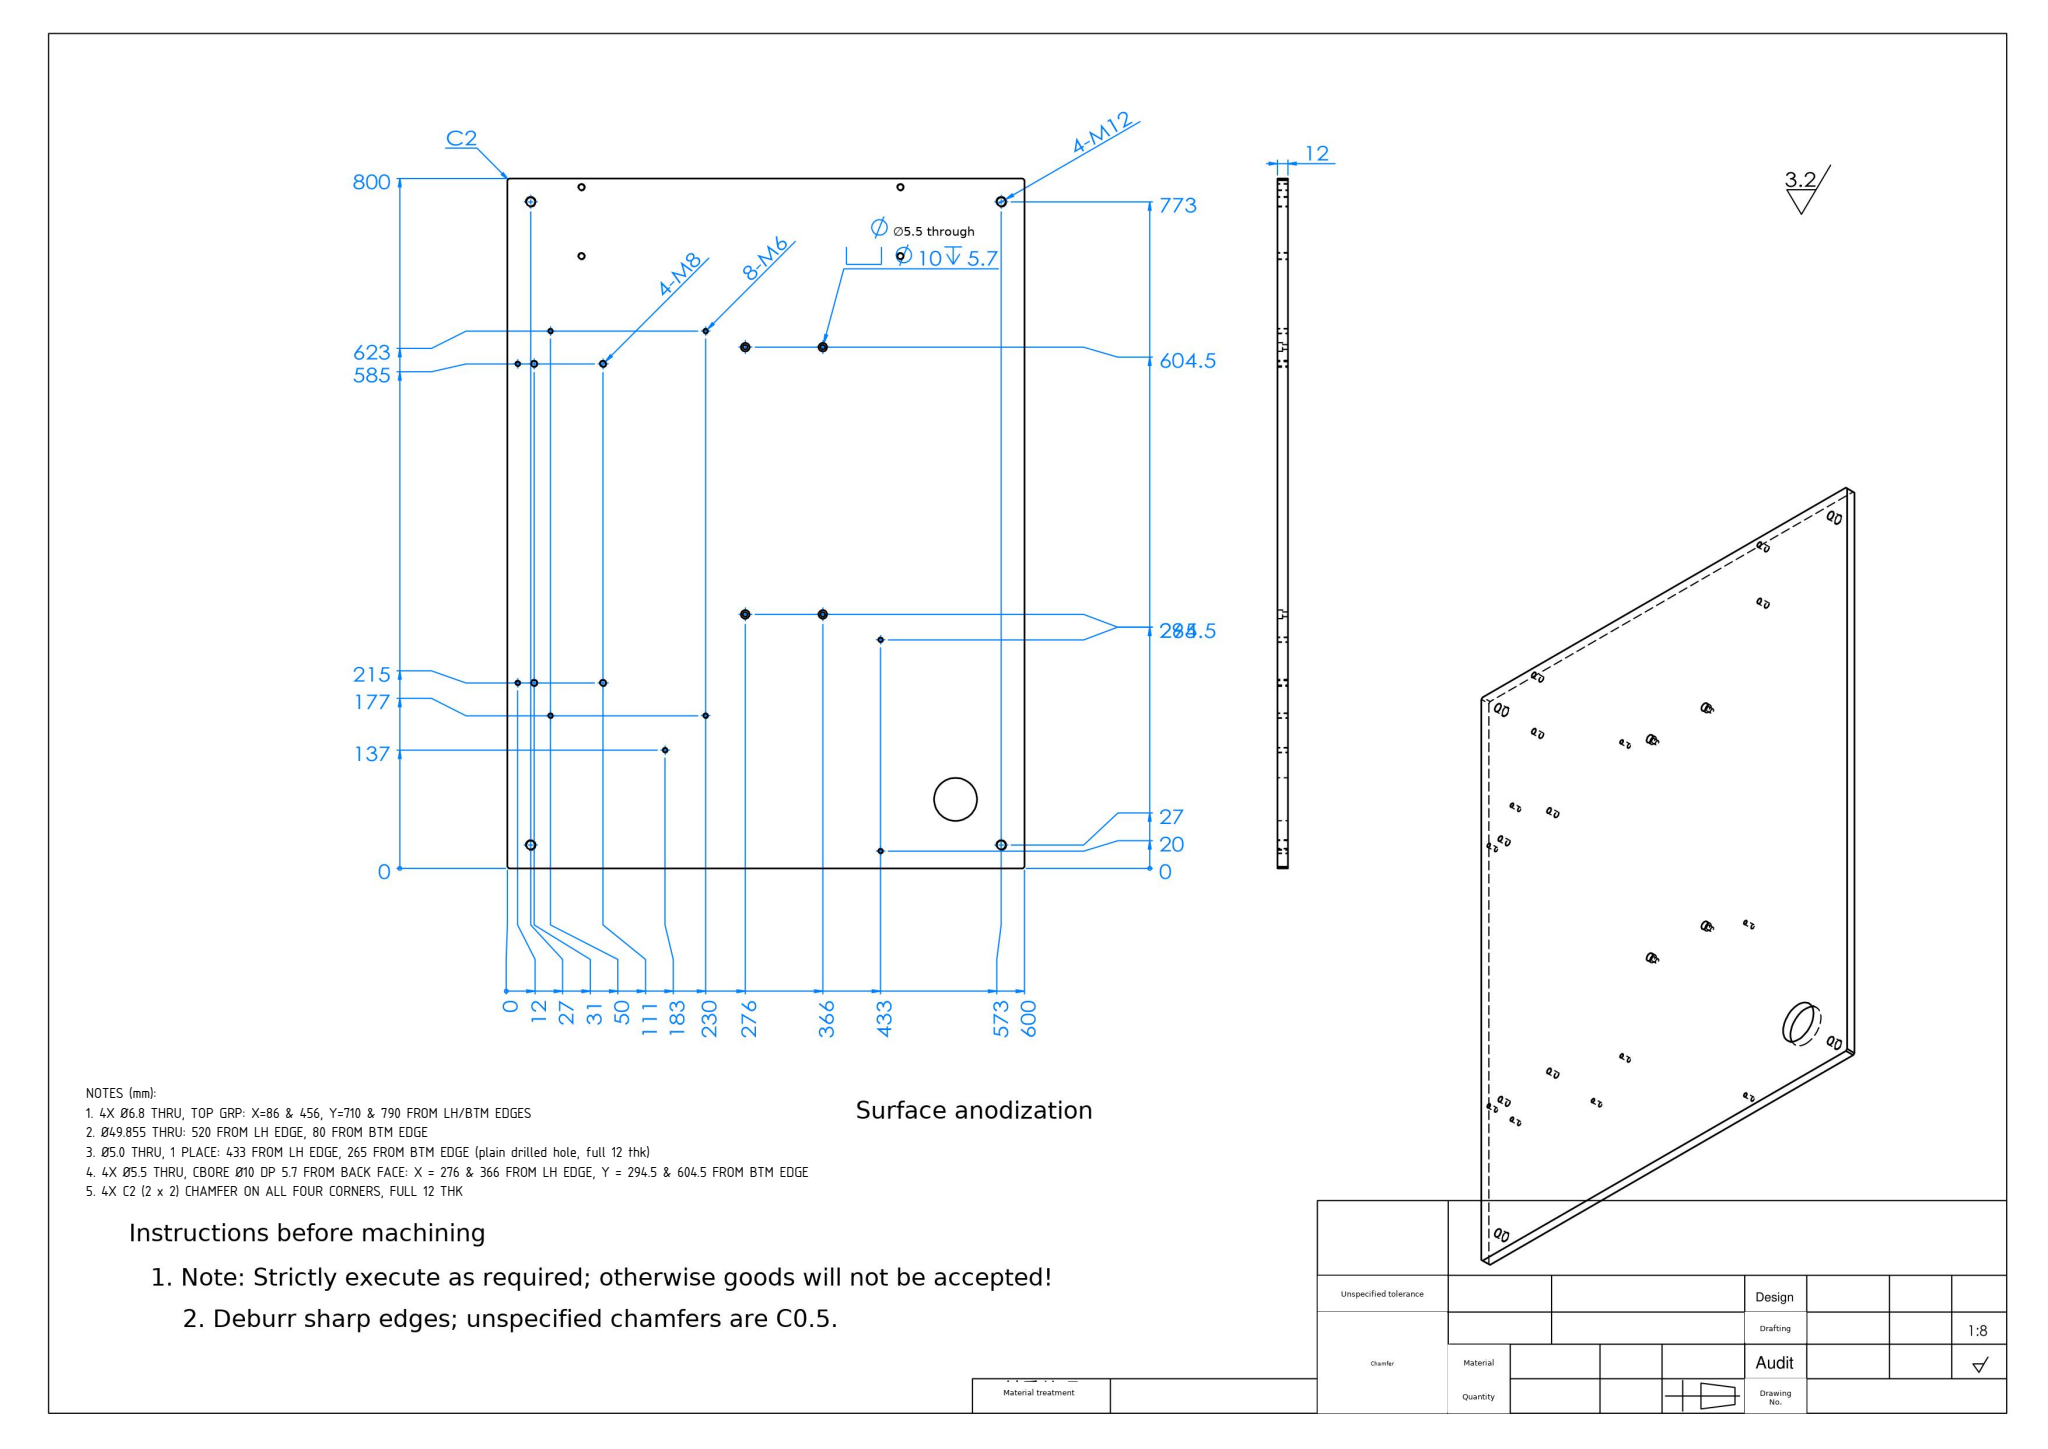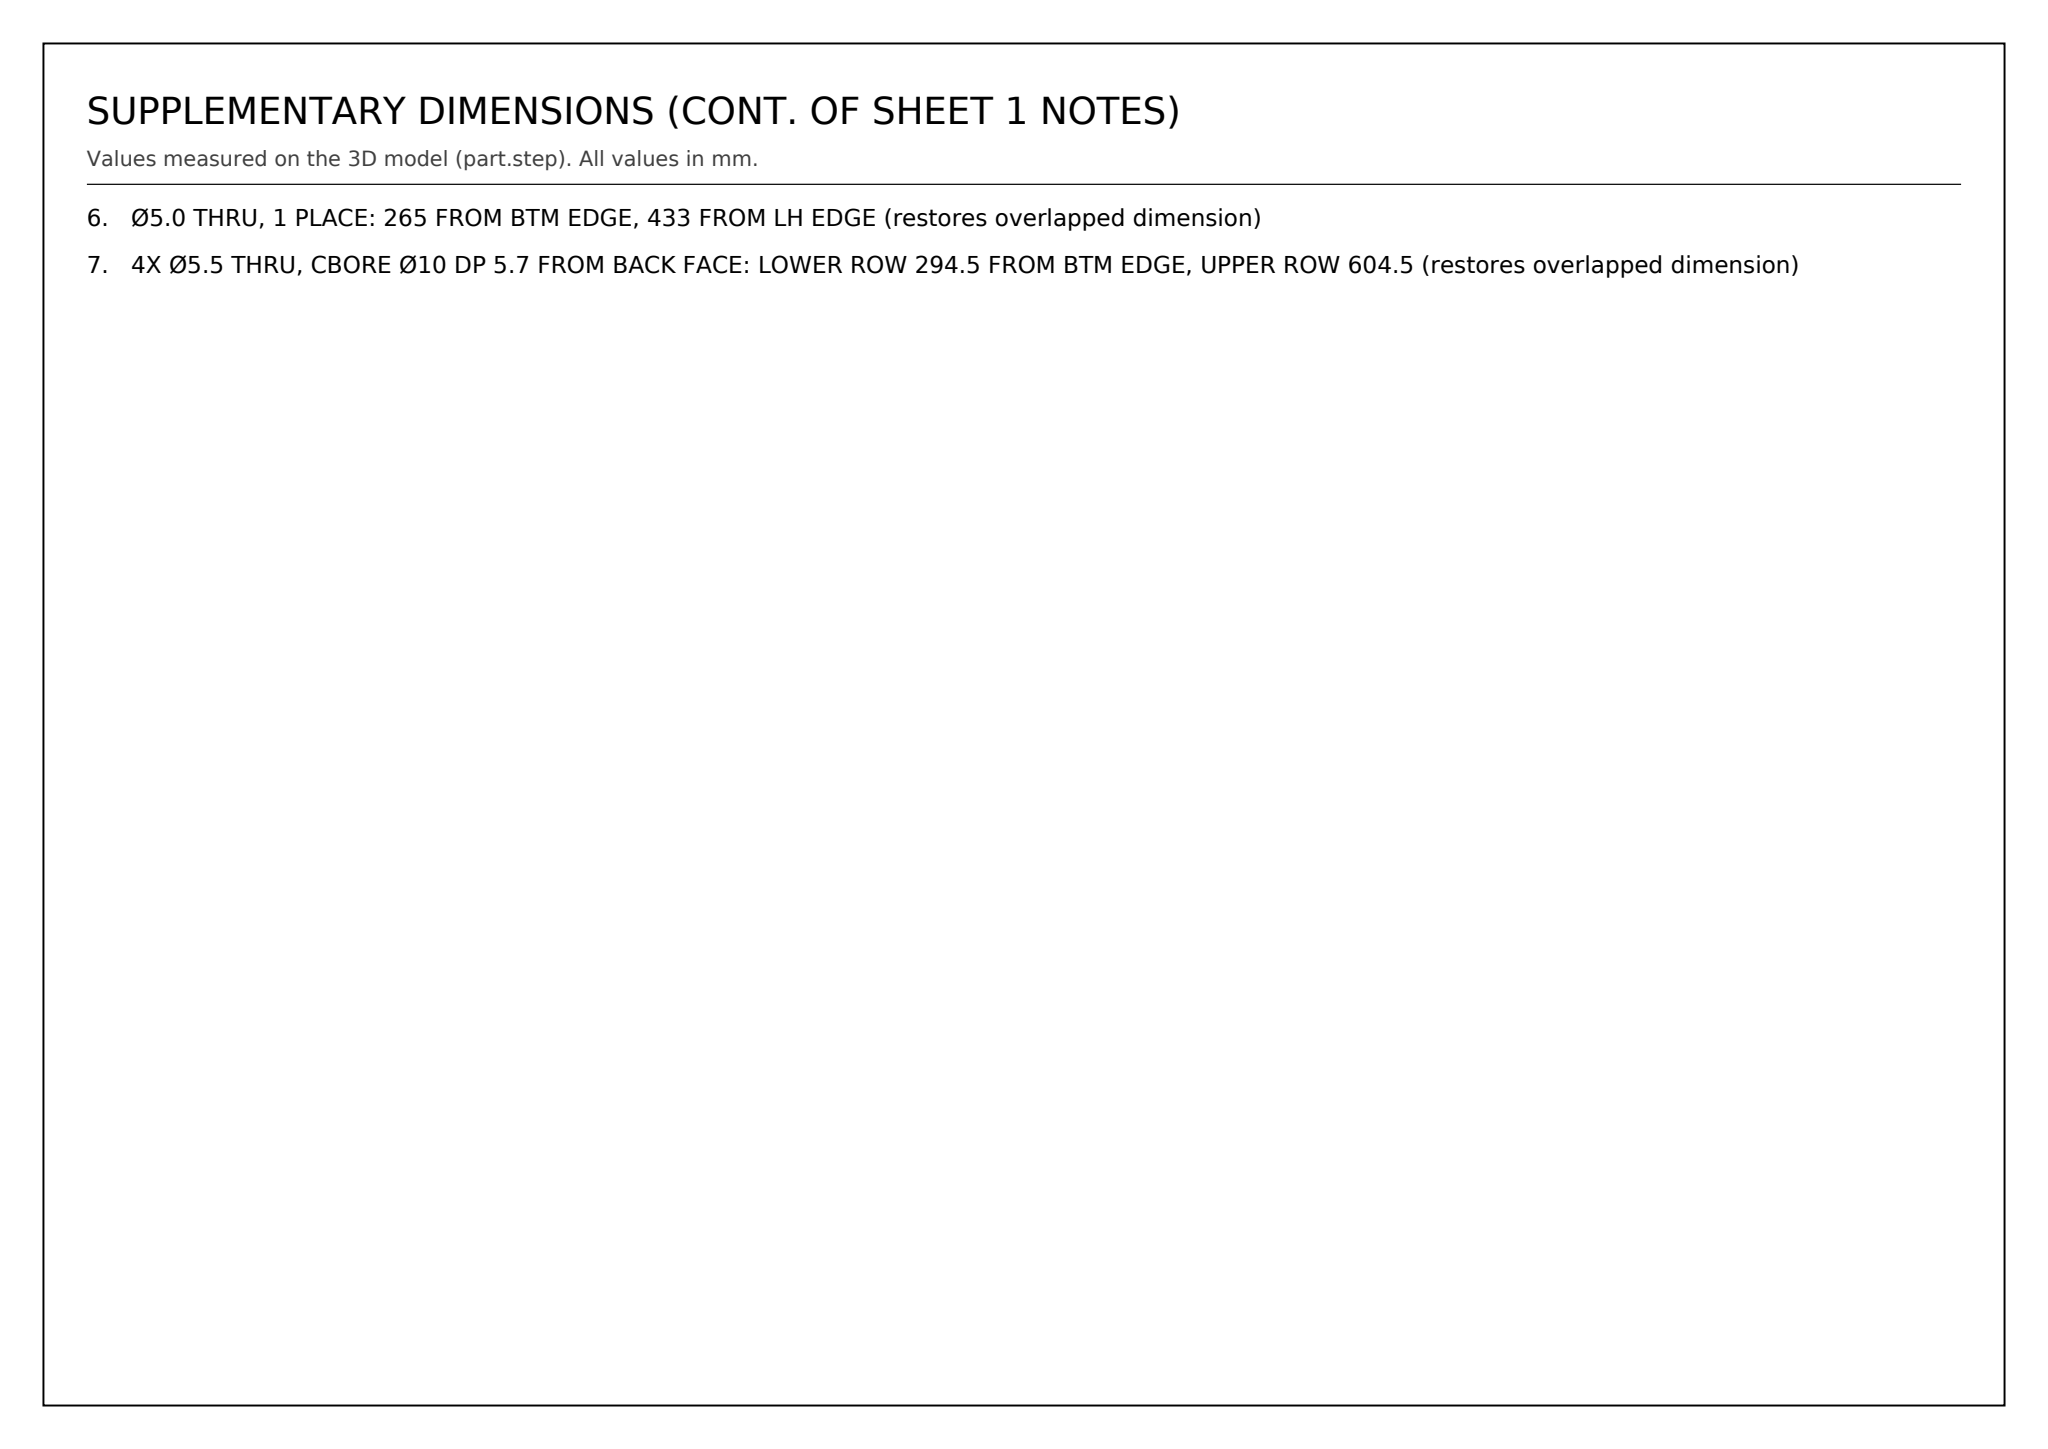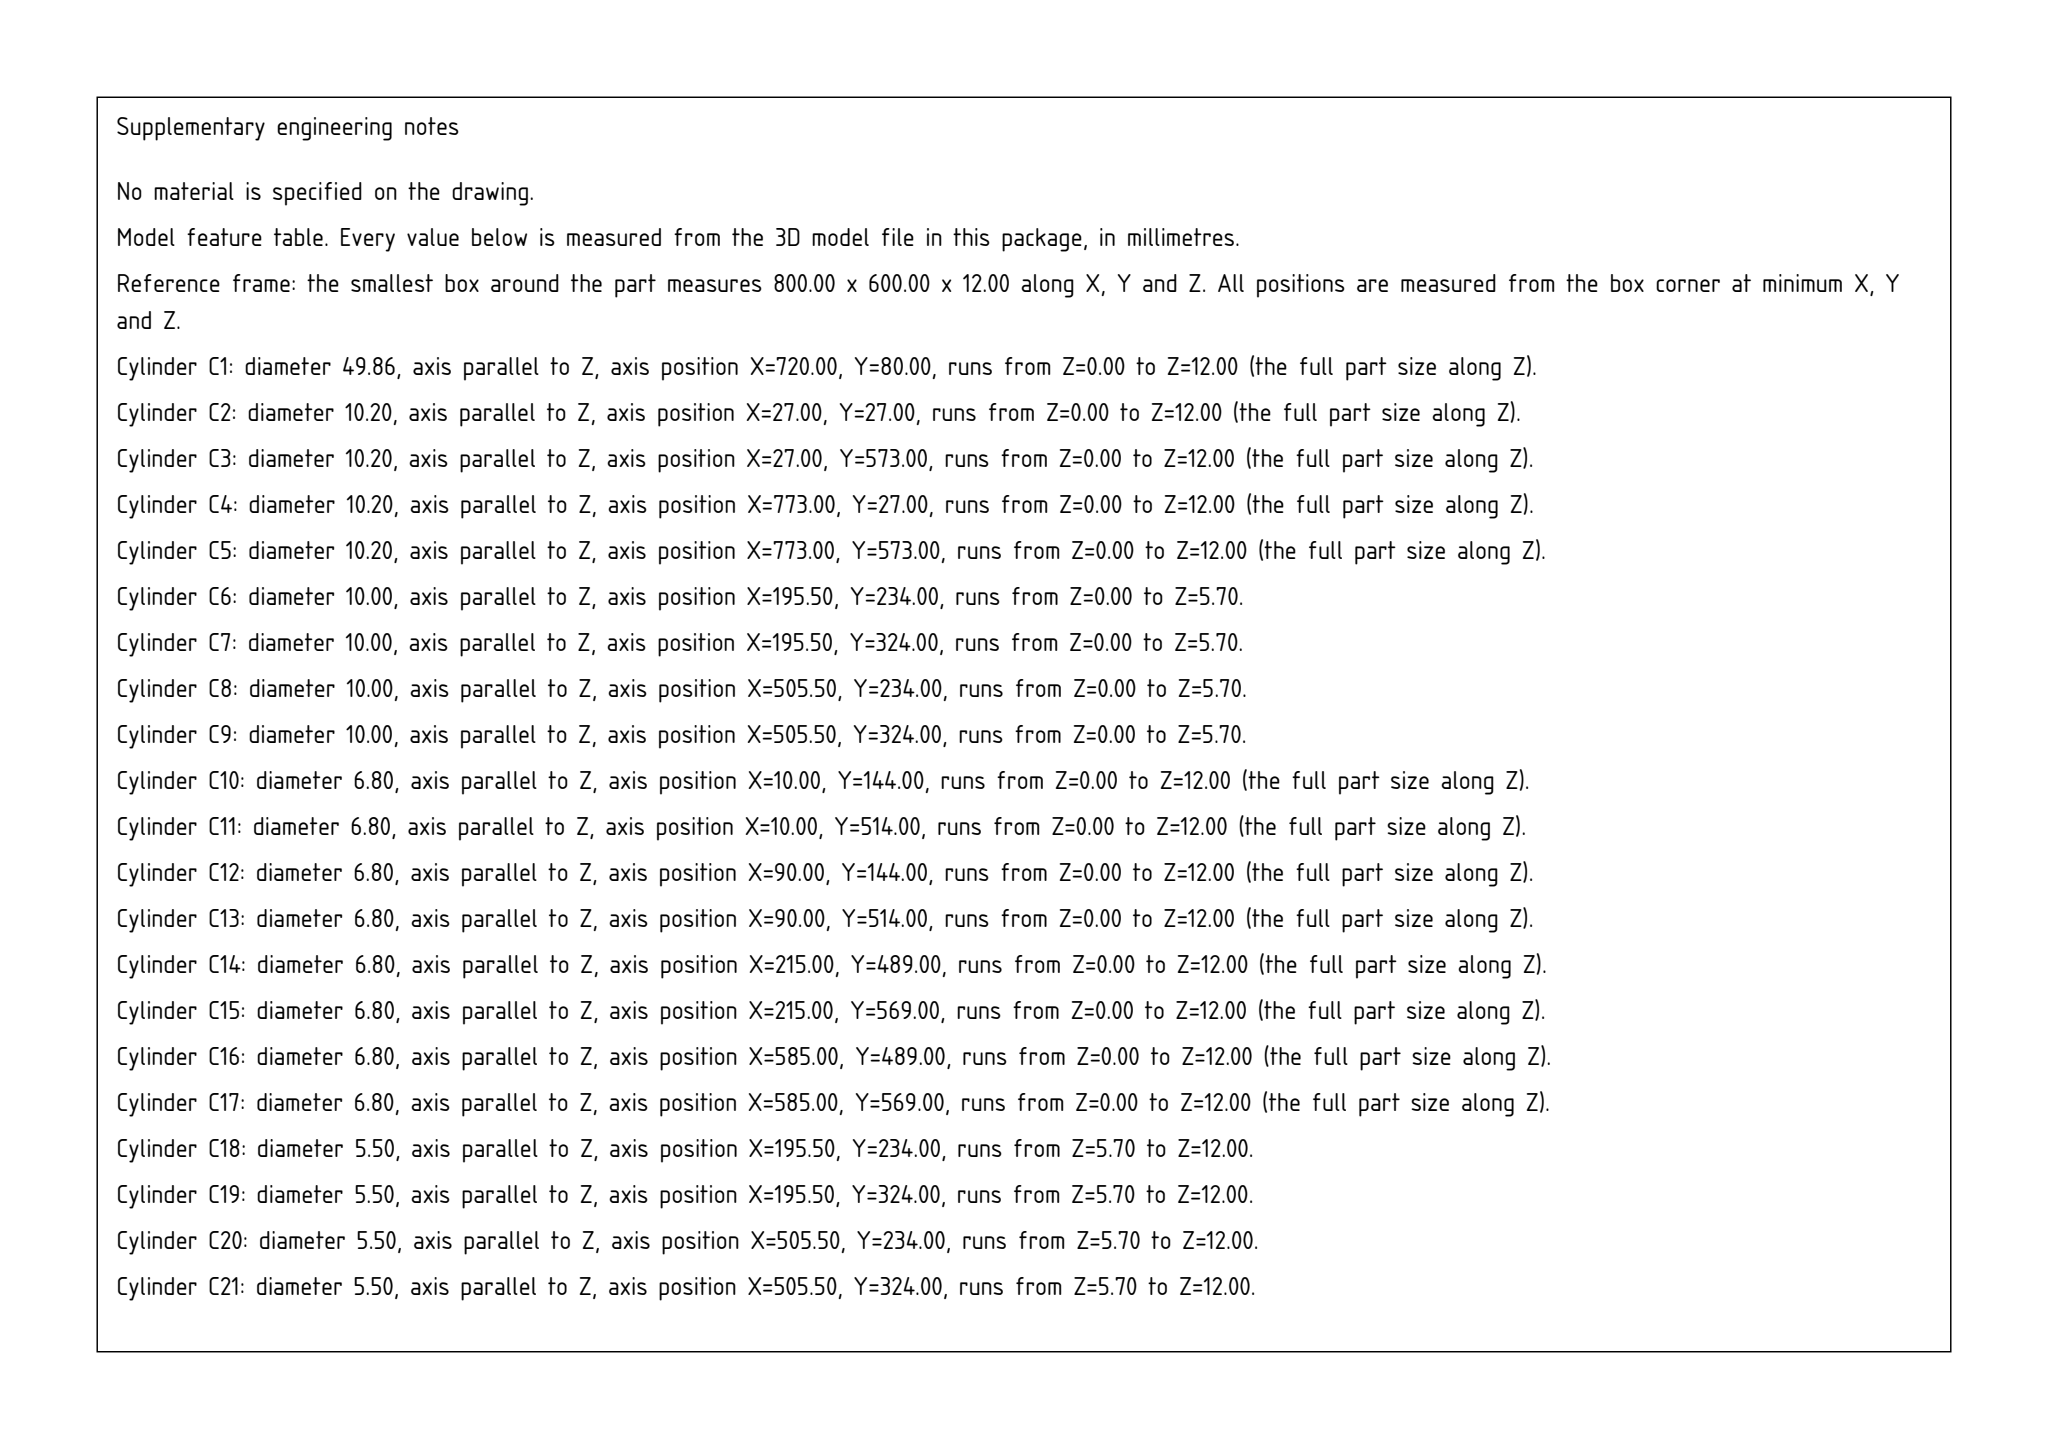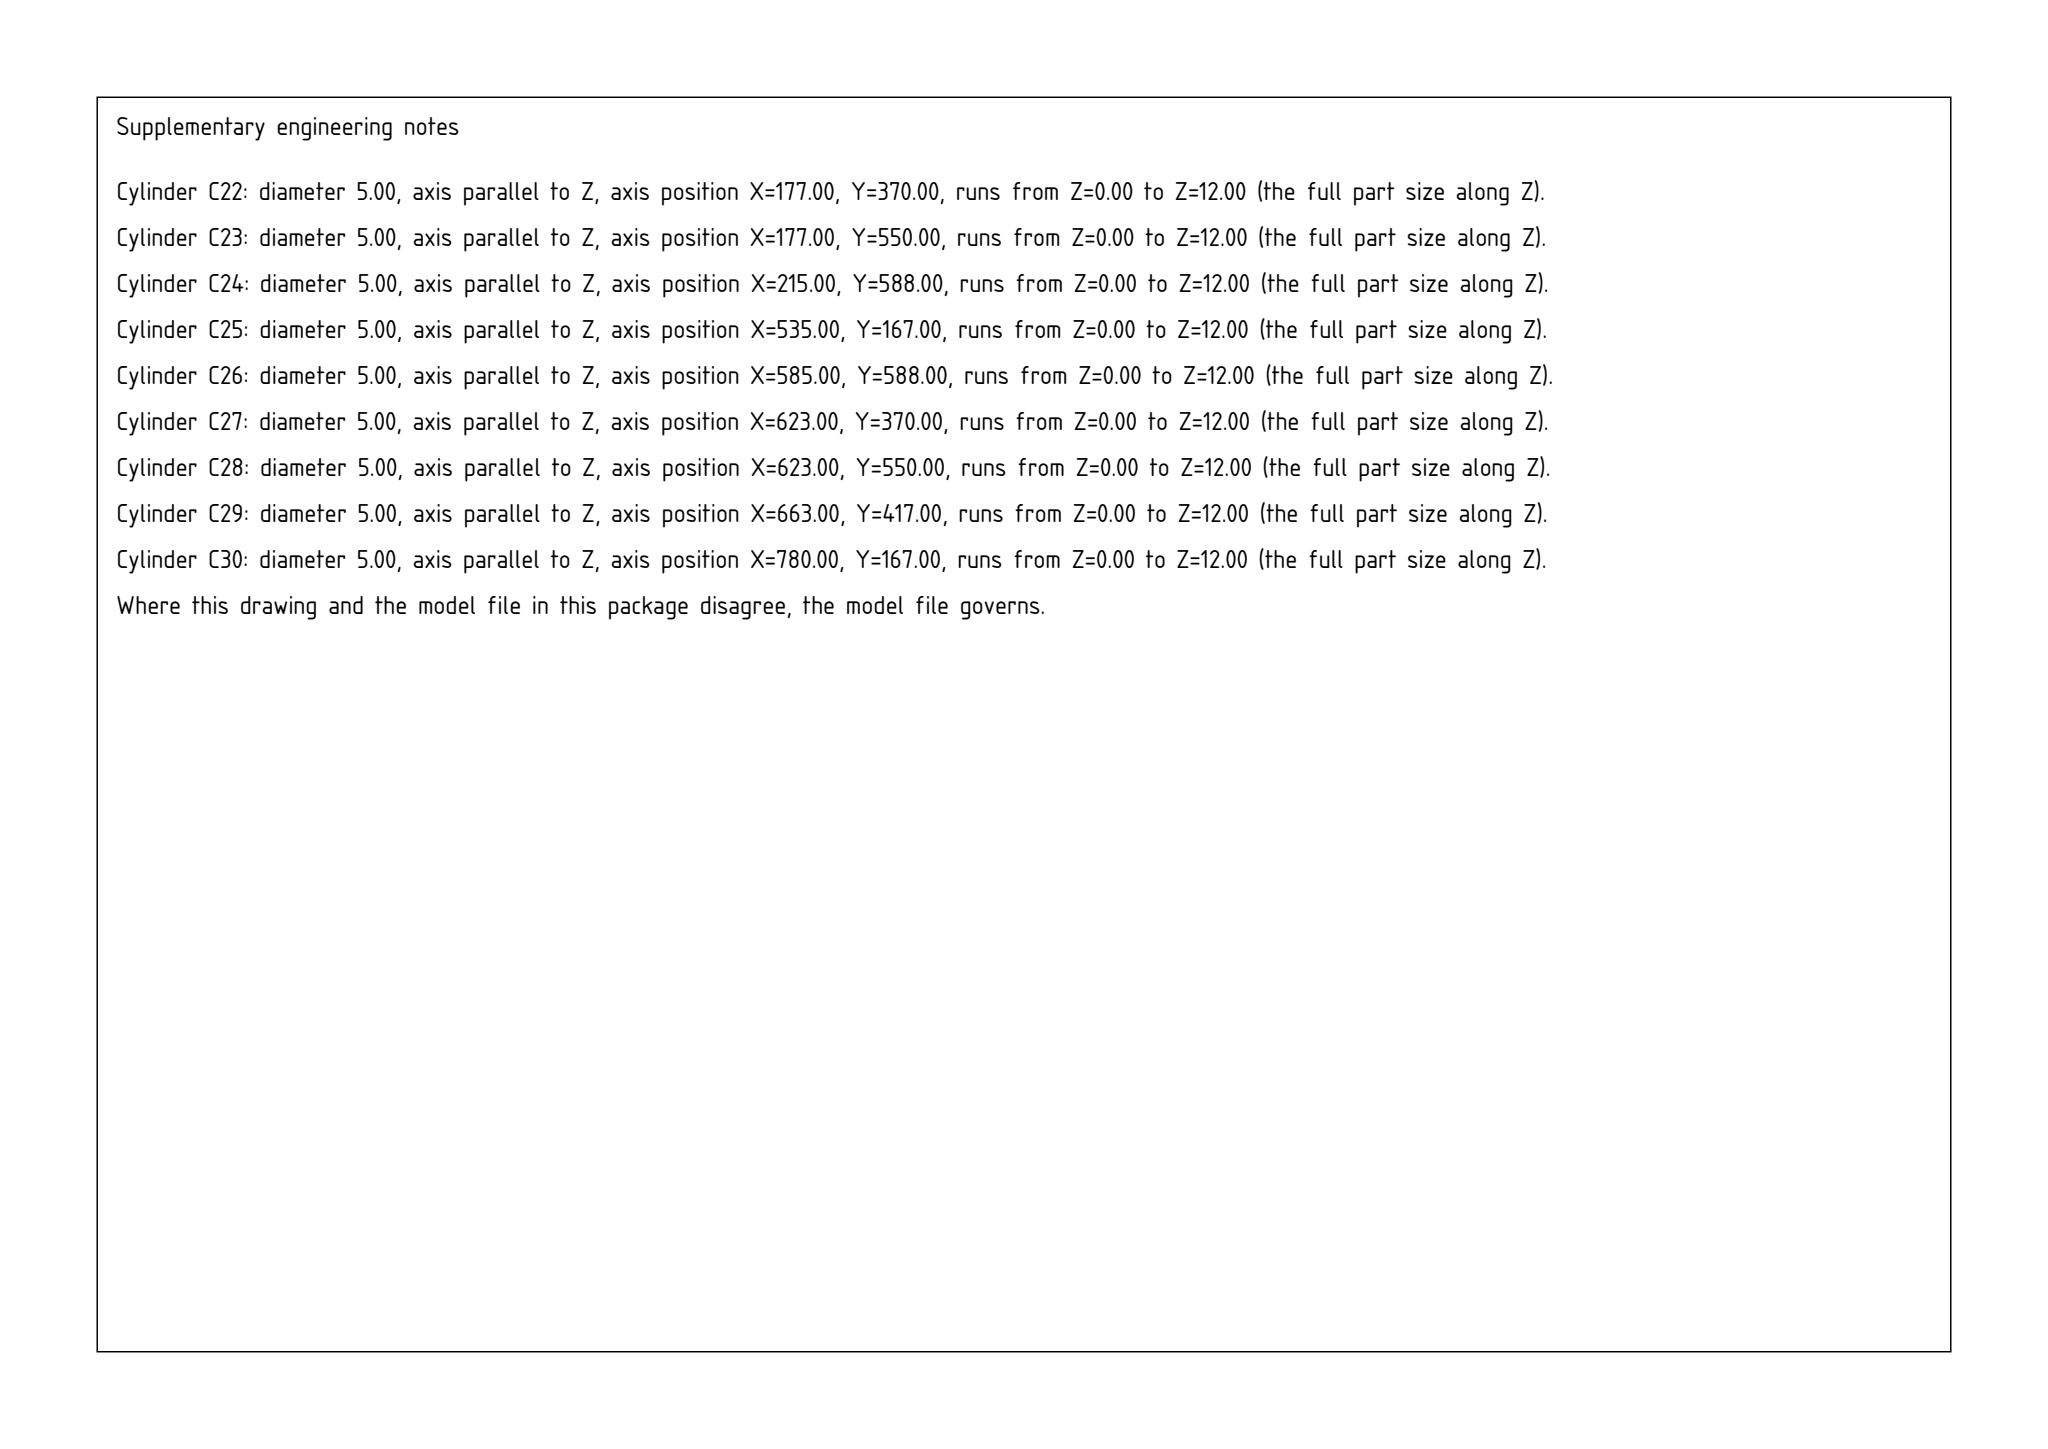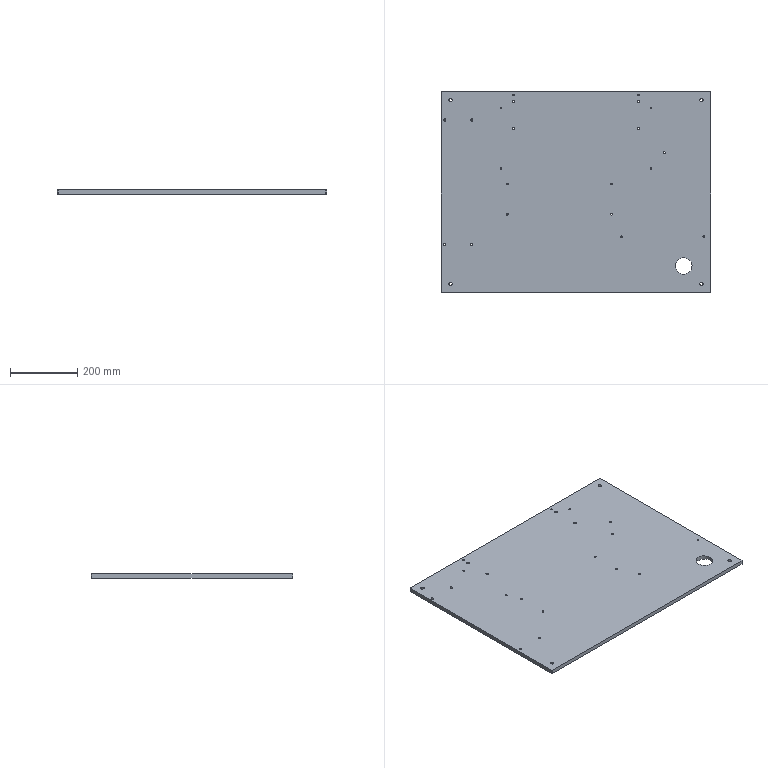Part | SolidWorks | mm | 1 solid | 74 faces | box 800 x 600 x 12 mm | volume 5724560 mm3 | cylinder 60 | plane 14 | commonest cylinder face diameters 5 x18 6.8 x16 10.2 x8 10 x8 5.5 x8 49.855 x2
Drawing notes:
4X Ø6.8 THRU, TOP GRP: X=86 & 456, Y=710 & 790 FROM LH/BTM EDGES | from the solid: dia 6.8 z-holes (10,144)(10,514)(90,144)(90,514), len 12 = thru; X=600-Y_m, Y=800-X_m
Ø49.855 THRU: 520 FROM LH EDGE, 80 FROM BTM EDGE | from the solid: cyl dia 49.855, axis z, pos (720,80), len 12 = thru; X=600-80=520, Y=800-720=80
Ø5.0 THRU, 1 PLACE: 433 FROM LH EDGE, 265 FROM BTM EDGE (plain drilled hole, full 12 thk) | from the solid: cylinder kind hole/bore dia 5.0 axis z at [535.0, 167.0] from 0.0 to 12.0 (drawing X = 600 - y = 433, drawing Y = 800 - x = 265)
4X Ø5.5 THRU, CBORE Ø10 DP 5.7 FROM BACK FACE: X = 276 & 366 FROM LH EDGE, Y = 294.5 & 604.5 FROM BTM EDGE | from the solid: cylinders dia 10.0 axis z at [195.5,234.0], [195.5,324.0], [505.5,234.0], [505.5,324.0] from 0.0 to 5.7, with dia 5.5 continuing 5.7 to 12.0 (drawing X = 600 - y, drawing Y = 800 - x)
4X C2 (2 x 2) CHAMFER ON ALL FOUR CORNERS, FULL 12 THK | from the solid: inclined_planes: four 45deg faces, size [2.0, 2.0, 12.0] at bbox_from [0,0,0], [0,598,0], [798,0,0], [798,598,0]
Ø5.0 THRU, 1 PLACE: 265 FROM BTM EDGE, 433 FROM LH EDGE (restores overlapped dimension) | from the solid: cylinders: hole/bore dia 5.0, axis z at [535.0, 167.0], from 0.0 to 12.0 (800-535 = 265 from btm edge)
4X Ø5.5 THRU, CBORE Ø10 DP 5.7 FROM BACK FACE: LOWER ROW 294.5 FROM BTM EDGE, UPPER ROW 604.5 (restores overlapped dimension) | from the solid: cylinders: hole/bore dia 10.0 axis z at [505.5,234.0] and [505.5,324.0] from 0.0 to 5.7 (800-505.5 = 294.5); dia 10.0 at [195.5,234.0] and [195.5,324.0] (800-195.5 = 604.5)
build123d program:
from build123d import *

# Parameters (mm, degrees)
SKETCH1_W                                         = 800
SKETCH1_H                                         = 600
BOSS_EXTRUDE1_DEPTH                               = 6
CHAMFER1_SIZE                                     = 2
M6_TAPPED_HOLE1_D                                 = 5
M8_TAPPED_HOLE1_D                                 = 6.8
M6_TAPPED_HOLE2_D                                 = 5
HOLE_SIZE_ACCORDING_TO_HEXAGON_SOCKET_D           = 5.5
HOLE_SIZE_ACCORDING_TO_HEXAGON_SOCKET_CBORE_D     = 10
HOLE_SIZE_ACCORDING_TO_HEXAGON_SOCKET_CBORE_DEPTH = 5.7
M12_TAPPED_HOLE1_D                                = 10.2
SKETCH16_R                                        = 24.928
CUT_EXTRUDE1_DEPTH                                = 20
M8_TAPPED_HOLE2_D                                 = 6.8


with BuildPart() as part:
    # Sketch1 → Boss-Extrude1 (new, symmetric)
    with BuildSketch(Plane.XY):
        Rectangle(SKETCH1_W, SKETCH1_H)
    extrude(amount=BOSS_EXTRUDE1_DEPTH, both=True)

    # Chamfer1
    chamfer1_edges = [part.edges().sort_by_distance(p)[0] for p in [
        (400, -300, 0),
        (-400, -300, 0),
        (-400, 300, 0),
        (400, 300, 0),
    ]]
    chamfer(chamfer1_edges, length=CHAMFER1_SIZE)

    # M6 Tapped Hole1 (through all)
    with Locations(Plane.XY.offset(6)):
        with Locations((-223, 70), (-223, 250), (-185, 288), (185, 288), (223, 250), (223, 70)):
            Hole(M6_TAPPED_HOLE1_D / 2)

    # M8 Tapped Hole1 (through all)
    with Locations(Plane.XY.offset(6)):
        with Locations((-185, 269), (-185, 189), (185, 269), (185, 189)):
            Hole(M8_TAPPED_HOLE1_D / 2)

    # M6 Tapped Hole2 (through all)
    with Locations(Plane.XY.offset(6)):
        with Locations((263, 117), (135, -133), (380, -133)):
            Hole(M6_TAPPED_HOLE2_D / 2)

    # Hole Size _ according to_ Hexagon Socket (through all)
    with Locations(Plane(origin=(0, 0, -6), x_dir=(-1, 0, 0), z_dir=(0, 0, -1))):
        with Locations((204.5, -66), (204.5, 24), (-105.5, 24), (-105.5, -66)):
            CounterBoreHole(HOLE_SIZE_ACCORDING_TO_HEXAGON_SOCKET_D / 2, HOLE_SIZE_ACCORDING_TO_HEXAGON_SOCKET_CBORE_D / 2, HOLE_SIZE_ACCORDING_TO_HEXAGON_SOCKET_CBORE_DEPTH)

    # M12 Tapped Hole1 (through all)
    with Locations(Plane.XY.offset(6)):
        with Locations((-373, -273), (373, -273), (373, 273), (-373, 273)):
            Hole(M12_TAPPED_HOLE1_D / 2)

    # Sketch16 → Cut-Extrude1 (cut)
    with BuildSketch(Plane.XY.offset(6)):
        with Locations((320, -220)):
            Circle(SKETCH16_R)
    extrude(amount=-CUT_EXTRUDE1_DEPTH, mode=Mode.SUBTRACT)

    # M8 Tapped Hole2 (through all)
    with Locations(Plane.XY.offset(6)):
        with Locations((-390, 214), (-310, 214), (-390, -156), (-310, -156)):
            Hole(M8_TAPPED_HOLE2_D / 2)


solid = part.part